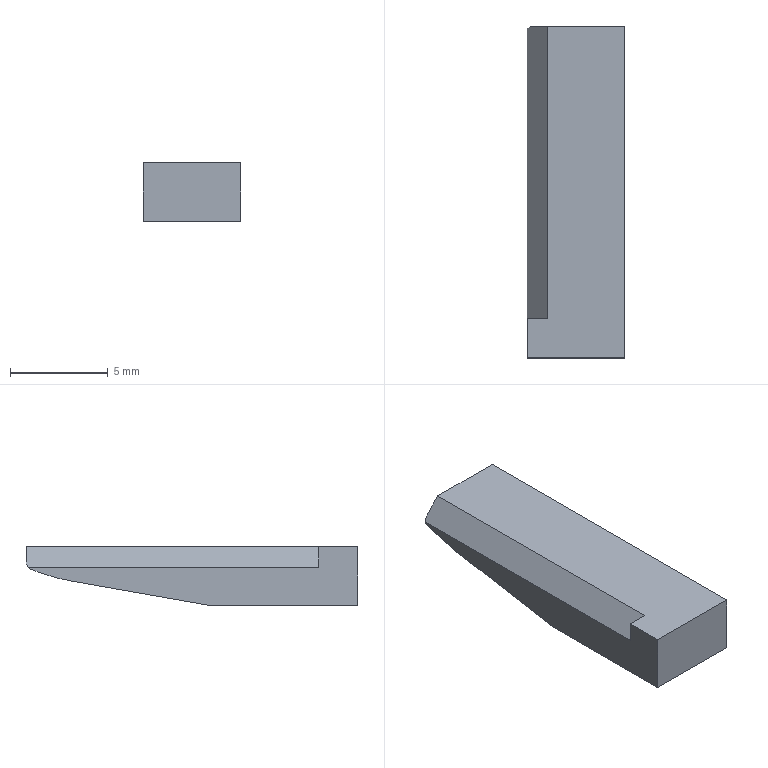Component | SolidWorks | 04LowerMaterialReceivingSwingAngleAssembly(3920)-1_04LowerMaterialReceivingDieAssembly(3920)-1_H2020022-0446-1(3920)-2 | 1 solid | 12 faces | box 5 x 17 x 3 mm | volume 207 mm3 | plane 10 | cylinder 2 | commonest cylinder face diameters 20 x1 1 x1 | material 45#Steel
build123d program:
from build123d import *

# Parameters (mm, degrees)
SKETCH1_W           = 5
SKETCH1_H           = 3
BOSS_EXTRUDE1_DEPTH = 17
CUT_EXTRUDE1_DEPTH  = 18.972
CUT_EXTRUDE2_DEPTH  = 18.972
FILLET2_R           = 10
FILLET3_R           = 0.5
CUT_EXTRUDE3_DEPTH  = 15


with BuildPart() as part:
    # Sketch1 → Boss-Extrude1 (new body)
    with BuildSketch(Plane(origin=(0, 0, 0), x_dir=(1, 0, 0), z_dir=(0, 1, 0))):
        with Locations((2.5, 1.5)):
            Rectangle(SKETCH1_W, SKETCH1_H)
    extrude(amount=BOSS_EXTRUDE1_DEPTH)

    # Sketch2 → Cut-Extrude1 (cut, through all)
    with BuildSketch(Plane.ZY):
        Polygon((-3, 7.65), (-1.351, 17), (-3, 17), align=None)
    extrude(amount=-CUT_EXTRUDE1_DEPTH, mode=Mode.SUBTRACT)

    # Sketch3 → Cut-Extrude2 (cut, through all)
    with BuildSketch(Plane.ZY):
        Polygon((-1.616, 15.5), (-1.07, 17), (-1.351, 17), align=None)
    extrude(amount=-CUT_EXTRUDE2_DEPTH, mode=Mode.SUBTRACT)

    # Fillet2
    fillet2_edges = [part.edges().sort_by_distance(p)[0] for p in [
        (2.5, 15.5, -1.616),
    ]]
    fillet(fillet2_edges, radius=FILLET2_R)

    # Fillet3
    fillet3_edges = [part.edges().sort_by_distance(p)[0] for p in [
        (2.5, 17, -1.07),
    ]]
    fillet(fillet3_edges, radius=FILLET3_R)

    # Sketch4 → Cut-Extrude3 (cut)
    with BuildSketch(Plane(origin=(0, 17, 0), x_dir=(1, 0, 0), z_dir=(0, 1, 0))):
        Polygon((0, 0), (0, 1.05), (1.05, 0), align=None)
    extrude(amount=-CUT_EXTRUDE3_DEPTH, mode=Mode.SUBTRACT)


solid = part.part

# Placed as in the assembly
solid = solid.moved(Location((-2.459, 271.013, 299.909), (0, 0, 0)))
STEP:
#1=COLOUR_RGB('',0.7922,0.8196,0.9333);
#2=FILL_AREA_STYLE_COLOUR('',#1);
#3=FILL_AREA_STYLE('',(#2));
#4=SURFACE_STYLE_FILL_AREA(#3);
#5=SURFACE_SIDE_STYLE('',(#4));
#6=SURFACE_STYLE_USAGE(.BOTH.,#5);
#7=PRESENTATION_STYLE_ASSIGNMENT((#6));
#8=CARTESIAN_POINT('',(-0.09682,10.749,11.766));
#9=VERTEX_POINT('',#8);
#10=CARTESIAN_POINT('',(-0.09682,10.749,11.807));
#11=VERTEX_POINT('',#10);
#12=CARTESIAN_POINT('',(-0.09682,10.749,11.807));
#13=DIRECTION('',(0.,0.,1.));
#14=VECTOR('',#13,39.37);
#15=LINE('',#12,#14);
#16=EDGE_CURVE('',#9,#11,#15,.T.);
#17=ORIENTED_EDGE('',*,*,#16,.F.);
#18=CARTESIAN_POINT('',(-0.09682,11.334,11.766));
#19=VERTEX_POINT('',#18);
#20=CARTESIAN_POINT('',(-0.09682,10.749,11.766));
#21=DIRECTION('',(0.,1.,0.));
#22=VECTOR('',#21,39.37);
#23=LINE('',#20,#22);
#24=EDGE_CURVE('',#9,#19,#23,.T.);
#25=ORIENTED_EDGE('',*,*,#24,.T.);
#26=CARTESIAN_POINT('',(-0.09682,11.326,11.761));
#27=VERTEX_POINT('',#26);
#28=CARTESIAN_POINT('',(-0.09682,11.319,11.779));
#29=DIRECTION('',(-1.,0.,0.));
#30=DIRECTION('',(0.,0.,-1.));
#31=AXIS2_PLACEMENT_3D('',#28,#29,#30);
#32=CIRCLE('',#31,0.01969);
#33=EDGE_CURVE('',#19,#27,#32,.T.);
#34=ORIENTED_EDGE('',*,*,#33,.T.);
#35=CARTESIAN_POINT('',(-0.09682,11.312,11.756));
#36=VERTEX_POINT('',#35);
#37=CARTESIAN_POINT('',(-0.09682,11.28,11.744));
#38=DIRECTION('',(0.,0.9397,0.342));
#39=VECTOR('',#38,39.37);
#40=LINE('',#37,#39);
#41=EDGE_CURVE('',#36,#27,#40,.T.);
#42=ORIENTED_EDGE('',*,*,#41,.F.);
#43=CARTESIAN_POINT('',(-0.09682,11.246,11.738));
#44=VERTEX_POINT('',#43);
#45=CARTESIAN_POINT('',(-0.09682,11.178,12.126));
#46=DIRECTION('',(-1.,0.,0.));
#47=DIRECTION('',(0.,-0.,-1.));
#48=AXIS2_PLACEMENT_3D('',#45,#46,#47);
#49=CIRCLE('',#48,0.3937);
#50=EDGE_CURVE('',#36,#44,#49,.T.);
#51=ORIENTED_EDGE('',*,*,#50,.T.);
#52=CARTESIAN_POINT('',(-0.09682,10.971,11.689));
#53=VERTEX_POINT('',#52);
#54=CARTESIAN_POINT('',(-0.09682,10.971,11.689));
#55=DIRECTION('',(0.,0.9848,0.1736));
#56=VECTOR('',#55,39.37);
#57=LINE('',#54,#56);
#58=EDGE_CURVE('',#53,#44,#57,.T.);
#59=ORIENTED_EDGE('',*,*,#58,.F.);
#60=CARTESIAN_POINT('',(-0.09682,10.67,11.689));
#61=VERTEX_POINT('',#60);
#62=CARTESIAN_POINT('',(-0.09682,11.339,11.689));
#63=DIRECTION('',(0.,-1.,0.));
#64=VECTOR('',#63,39.37);
#65=LINE('',#62,#64);
#66=EDGE_CURVE('',#53,#61,#65,.T.);
#67=ORIENTED_EDGE('',*,*,#66,.T.);
#68=CARTESIAN_POINT('',(-0.09682,10.67,11.807));
#69=VERTEX_POINT('',#68);
#70=CARTESIAN_POINT('',(-0.09682,10.67,11.807));
#71=DIRECTION('',(0.,0.,1.));
#72=VECTOR('',#71,39.37);
#73=LINE('',#70,#72);
#74=EDGE_CURVE('',#61,#69,#73,.T.);
#75=ORIENTED_EDGE('',*,*,#74,.T.);
#76=CARTESIAN_POINT('',(-0.09682,11.339,11.807));
#77=DIRECTION('',(0.,-1.,0.));
#78=VECTOR('',#77,39.37);
#79=LINE('',#76,#78);
#80=EDGE_CURVE('',#11,#69,#79,.T.);
#81=ORIENTED_EDGE('',*,*,#80,.F.);
#82=EDGE_LOOP('',(#17,#25,#34,#42,#51,#59,#67,#75,#81));
#83=FACE_OUTER_BOUND('',#82,.T.);
#84=CARTESIAN_POINT('',(-0.09682,11.339,11.807));
#85=DIRECTION('',(1.,0.,0.));
#86=DIRECTION('',(0.,0.,-1.));
#87=AXIS2_PLACEMENT_3D('',#84,#85,#86);
#88=PLANE('',#87);
#89=ADVANCED_FACE('',(#83),#88,.F.);
#90=CARTESIAN_POINT('',(-0.05548,11.339,11.807));
#91=VERTEX_POINT('',#90);
#92=CARTESIAN_POINT('',(0.1,11.339,11.807));
#93=VERTEX_POINT('',#92);
#94=CARTESIAN_POINT('',(-0.09682,11.339,11.807));
#95=DIRECTION('',(1.,0.,0.));
#96=VECTOR('',#95,39.37);
#97=LINE('',#94,#96);
#98=EDGE_CURVE('',#91,#93,#97,.T.);
#99=ORIENTED_EDGE('',*,*,#98,.F.);
#100=CARTESIAN_POINT('',(-0.05548,10.749,11.807));
#101=VERTEX_POINT('',#100);
#102=CARTESIAN_POINT('',(-0.05548,10.749,11.807));
#103=DIRECTION('',(0.,1.,0.));
#104=VECTOR('',#103,39.37);
#105=LINE('',#102,#104);
#106=EDGE_CURVE('',#101,#91,#105,.T.);
#107=ORIENTED_EDGE('',*,*,#106,.F.);
#108=CARTESIAN_POINT('',(-0.05548,10.749,11.807));
#109=DIRECTION('',(1.,0.,0.));
#110=VECTOR('',#109,39.37);
#111=LINE('',#108,#110);
#112=EDGE_CURVE('',#11,#101,#111,.T.);
#113=ORIENTED_EDGE('',*,*,#112,.F.);
#114=ORIENTED_EDGE('',*,*,#80,.T.);
#115=CARTESIAN_POINT('',(0.1,10.67,11.807));
#116=VERTEX_POINT('',#115);
#117=CARTESIAN_POINT('',(-0.09682,10.67,11.807));
#118=DIRECTION('',(1.,0.,0.));
#119=VECTOR('',#118,39.37);
#120=LINE('',#117,#119);
#121=EDGE_CURVE('',#69,#116,#120,.T.);
#122=ORIENTED_EDGE('',*,*,#121,.T.);
#123=CARTESIAN_POINT('',(0.1,11.339,11.807));
#124=DIRECTION('',(0.,-1.,0.));
#125=VECTOR('',#124,39.37);
#126=LINE('',#123,#125);
#127=EDGE_CURVE('',#93,#116,#126,.T.);
#128=ORIENTED_EDGE('',*,*,#127,.F.);
#129=EDGE_LOOP('',(#99,#107,#113,#114,#122,#128));
#130=FACE_OUTER_BOUND('',#129,.T.);
#131=CARTESIAN_POINT('',(-0.09682,11.339,11.807));
#132=DIRECTION('',(0.,0.,-1.));
#133=DIRECTION('',(-1.,0.,0.));
#134=AXIS2_PLACEMENT_3D('',#131,#132,#133);
#135=PLANE('',#134);
#136=ADVANCED_FACE('',(#130),#135,.F.);
#137=CARTESIAN_POINT('',(0.1,11.312,11.756));
#138=VERTEX_POINT('',#137);
#139=CARTESIAN_POINT('',(0.1,11.326,11.761));
#140=VERTEX_POINT('',#139);
#141=CARTESIAN_POINT('',(0.1,11.28,11.744));
#142=DIRECTION('',(0.,0.9397,0.342));
#143=VECTOR('',#142,39.37);
#144=LINE('',#141,#143);
#145=EDGE_CURVE('',#138,#140,#144,.T.);
#146=ORIENTED_EDGE('',*,*,#145,.T.);
#147=CARTESIAN_POINT('',(0.1,11.339,11.779));
#148=VERTEX_POINT('',#147);
#149=CARTESIAN_POINT('',(0.1,11.319,11.779));
#150=DIRECTION('',(1.,0.,0.));
#151=DIRECTION('',(0.,0.,1.));
#152=AXIS2_PLACEMENT_3D('',#149,#150,#151);
#153=CIRCLE('',#152,0.01969);
#154=EDGE_CURVE('',#140,#148,#153,.T.);
#155=ORIENTED_EDGE('',*,*,#154,.T.);
#156=CARTESIAN_POINT('',(0.1,11.339,11.807));
#157=DIRECTION('',(0.,0.,-1.));
#158=VECTOR('',#157,39.37);
#159=LINE('',#156,#158);
#160=EDGE_CURVE('',#93,#148,#159,.T.);
#161=ORIENTED_EDGE('',*,*,#160,.F.);
#162=ORIENTED_EDGE('',*,*,#127,.T.);
#163=CARTESIAN_POINT('',(0.1,10.67,11.689));
#164=VERTEX_POINT('',#163);
#165=CARTESIAN_POINT('',(0.1,10.67,11.807));
#166=DIRECTION('',(0.,0.,-1.));
#167=VECTOR('',#166,39.37);
#168=LINE('',#165,#167);
#169=EDGE_CURVE('',#116,#164,#168,.T.);
#170=ORIENTED_EDGE('',*,*,#169,.T.);
#171=CARTESIAN_POINT('',(0.1,10.971,11.689));
#172=VERTEX_POINT('',#171);
#173=CARTESIAN_POINT('',(0.1,11.339,11.689));
#174=DIRECTION('',(0.,-1.,0.));
#175=VECTOR('',#174,39.37);
#176=LINE('',#173,#175);
#177=EDGE_CURVE('',#172,#164,#176,.T.);
#178=ORIENTED_EDGE('',*,*,#177,.F.);
#179=CARTESIAN_POINT('',(0.1,11.246,11.738));
#180=VERTEX_POINT('',#179);
#181=CARTESIAN_POINT('',(0.1,10.971,11.689));
#182=DIRECTION('',(0.,0.9848,0.1736));
#183=VECTOR('',#182,39.37);
#184=LINE('',#181,#183);
#185=EDGE_CURVE('',#172,#180,#184,.T.);
#186=ORIENTED_EDGE('',*,*,#185,.T.);
#187=CARTESIAN_POINT('',(0.1,11.178,12.126));
#188=DIRECTION('',(1.,0.,0.));
#189=DIRECTION('',(0.,0.,1.));
#190=AXIS2_PLACEMENT_3D('',#187,#188,#189);
#191=CIRCLE('',#190,0.3937);
#192=EDGE_CURVE('',#180,#138,#191,.T.);
#193=ORIENTED_EDGE('',*,*,#192,.T.);
#194=EDGE_LOOP('',(#146,#155,#161,#162,#170,#178,#186,#193));
#195=FACE_OUTER_BOUND('',#194,.T.);
#196=CARTESIAN_POINT('',(0.1,11.339,11.807));
#197=DIRECTION('',(-1.,0.,0.));
#198=DIRECTION('',(0.,0.,1.));
#199=AXIS2_PLACEMENT_3D('',#196,#197,#198);
#200=PLANE('',#199);
#201=ADVANCED_FACE('',(#195),#200,.F.);
#202=ORIENTED_EDGE('',*,*,#66,.F.);
#203=CARTESIAN_POINT('',(0.1,10.971,11.689));
#204=DIRECTION('',(-1.,0.,0.));
#205=VECTOR('',#204,39.37);
#206=LINE('',#203,#205);
#207=EDGE_CURVE('',#172,#53,#206,.T.);
#208=ORIENTED_EDGE('',*,*,#207,.F.);
#209=ORIENTED_EDGE('',*,*,#177,.T.);
#210=CARTESIAN_POINT('',(-0.09682,10.67,11.689));
#211=DIRECTION('',(-1.,0.,0.));
#212=VECTOR('',#211,39.37);
#213=LINE('',#210,#212);
#214=EDGE_CURVE('',#164,#61,#213,.T.);
#215=ORIENTED_EDGE('',*,*,#214,.T.);
#216=EDGE_LOOP('',(#202,#208,#209,#215));
#217=FACE_OUTER_BOUND('',#216,.T.);
#218=CARTESIAN_POINT('',(-0.09682,11.339,11.689));
#219=DIRECTION('',(0.,0.,1.));
#220=DIRECTION('',(1.,0.,0.));
#221=AXIS2_PLACEMENT_3D('',#218,#219,#220);
#222=PLANE('',#221);
#223=ADVANCED_FACE('',(#217),#222,.F.);
#224=CARTESIAN_POINT('',(-0.08382,11.339,11.779));
#225=VERTEX_POINT('',#224);
#226=CARTESIAN_POINT('',(-0.09682,11.339,11.779));
#227=DIRECTION('',(-1.,0.,0.));
#228=VECTOR('',#227,39.37);
#229=LINE('',#226,#228);
#230=EDGE_CURVE('',#148,#225,#229,.T.);
#231=ORIENTED_EDGE('',*,*,#230,.T.);
#232=CARTESIAN_POINT('',(-0.09682,11.339,11.766));
#233=DIRECTION('',(-0.7071,0.,-0.7071));
#234=VECTOR('',#233,39.37);
#235=LINE('',#232,#234);
#236=EDGE_CURVE('',#91,#225,#235,.T.);
#237=ORIENTED_EDGE('',*,*,#236,.F.);
#238=ORIENTED_EDGE('',*,*,#98,.T.);
#239=ORIENTED_EDGE('',*,*,#160,.T.);
#240=EDGE_LOOP('',(#231,#237,#238,#239));
#241=FACE_OUTER_BOUND('',#240,.T.);
#242=CARTESIAN_POINT('',(-0.09682,11.339,11.807));
#243=DIRECTION('',(0.,-1.,0.));
#244=DIRECTION('',(0.,0.,-1.));
#245=AXIS2_PLACEMENT_3D('',#242,#243,#244);
#246=PLANE('',#245);
#247=ADVANCED_FACE('',(#241),#246,.F.);
#248=ORIENTED_EDGE('',*,*,#74,.F.);
#249=ORIENTED_EDGE('',*,*,#214,.F.);
#250=ORIENTED_EDGE('',*,*,#169,.F.);
#251=ORIENTED_EDGE('',*,*,#121,.F.);
#252=EDGE_LOOP('',(#248,#249,#250,#251));
#253=FACE_OUTER_BOUND('',#252,.T.);
#254=CARTESIAN_POINT('',(-0.09682,10.67,11.807));
#255=DIRECTION('',(0.,-1.,0.));
#256=DIRECTION('',(0.,0.,-1.));
#257=AXIS2_PLACEMENT_3D('',#254,#255,#256);
#258=PLANE('',#257);
#259=ADVANCED_FACE('',(#253),#258,.T.);
#260=ORIENTED_EDGE('',*,*,#58,.T.);
#261=CARTESIAN_POINT('',(0.1,11.246,11.738));
#262=DIRECTION('',(1.,0.,0.));
#263=VECTOR('',#262,39.37);
#264=LINE('',#261,#263);
#265=EDGE_CURVE('',#44,#180,#264,.T.);
#266=ORIENTED_EDGE('',*,*,#265,.T.);
#267=ORIENTED_EDGE('',*,*,#185,.F.);
#268=ORIENTED_EDGE('',*,*,#207,.T.);
#269=EDGE_LOOP('',(#260,#266,#267,#268));
#270=FACE_OUTER_BOUND('',#269,.T.);
#271=CARTESIAN_POINT('',(0.1,10.971,11.689));
#272=DIRECTION('',(0.,-0.1736,0.9848));
#273=DIRECTION('',(0.,-0.9848,-0.1736));
#274=AXIS2_PLACEMENT_3D('',#271,#272,#273);
#275=PLANE('',#274);
#276=ADVANCED_FACE('',(#270),#275,.F.);
#277=ORIENTED_EDGE('',*,*,#41,.T.);
#278=CARTESIAN_POINT('',(0.1,11.326,11.761));
#279=DIRECTION('',(1.,0.,0.));
#280=VECTOR('',#279,39.37);
#281=LINE('',#278,#280);
#282=EDGE_CURVE('',#27,#140,#281,.T.);
#283=ORIENTED_EDGE('',*,*,#282,.T.);
#284=ORIENTED_EDGE('',*,*,#145,.F.);
#285=CARTESIAN_POINT('',(0.1,11.312,11.756));
#286=DIRECTION('',(-1.,0.,0.));
#287=VECTOR('',#286,39.37);
#288=LINE('',#285,#287);
#289=EDGE_CURVE('',#138,#36,#288,.T.);
#290=ORIENTED_EDGE('',*,*,#289,.T.);
#291=EDGE_LOOP('',(#277,#283,#284,#290));
#292=FACE_OUTER_BOUND('',#291,.T.);
#293=CARTESIAN_POINT('',(0.1,11.28,11.744));
#294=DIRECTION('',(0.,-0.342,0.9397));
#295=DIRECTION('',(0.,-0.9397,-0.342));
#296=AXIS2_PLACEMENT_3D('',#293,#294,#295);
#297=PLANE('',#296);
#298=ADVANCED_FACE('',(#292),#297,.F.);
#299=ORIENTED_EDGE('',*,*,#192,.F.);
#300=ORIENTED_EDGE('',*,*,#265,.F.);
#301=ORIENTED_EDGE('',*,*,#50,.F.);
#302=ORIENTED_EDGE('',*,*,#289,.F.);
#303=EDGE_LOOP('',(#299,#300,#301,#302));
#304=FACE_OUTER_BOUND('',#303,.T.);
#305=CARTESIAN_POINT('',(0.1,11.178,12.126));
#306=DIRECTION('',(-1.,0.,0.));
#307=DIRECTION('',(0.,0.,1.));
#308=AXIS2_PLACEMENT_3D('',#305,#306,#307);
#309=CYLINDRICAL_SURFACE('',#308,0.3937);
#310=ADVANCED_FACE('',(#304),#309,.T.);
#311=CARTESIAN_POINT('',(-0.08382,11.339,11.779));
#312=CARTESIAN_POINT('',(-0.08866,11.339,11.774));
#313=CARTESIAN_POINT('',(-0.09319,11.337,11.77));
#314=CARTESIAN_POINT('',(-0.09682,11.334,11.766));
#315=(BOUNDED_CURVE()B_SPLINE_CURVE(3,(#311,#312,#313,#314),.UNSPECIFIED.,.F.,.T.)B_SPLINE_CURVE_WITH_KNOTS((4,4),(4.712,5.434),.UNSPECIFIED.)CURVE()GEOMETRIC_REPRESENTATION_ITEM()RATIONAL_B_SPLINE_CURVE((1.,0.9571,0.9571,1.))REPRESENTATION_ITEM(''));
#316=EDGE_CURVE('',#225,#19,#315,.T.);
#317=ORIENTED_EDGE('',*,*,#316,.F.);
#318=ORIENTED_EDGE('',*,*,#230,.F.);
#319=ORIENTED_EDGE('',*,*,#154,.F.);
#320=ORIENTED_EDGE('',*,*,#282,.F.);
#321=ORIENTED_EDGE('',*,*,#33,.F.);
#322=EDGE_LOOP('',(#317,#318,#319,#320,#321));
#323=FACE_OUTER_BOUND('',#322,.T.);
#324=CARTESIAN_POINT('',(-0.09682,11.319,11.779));
#325=DIRECTION('',(-1.,0.,0.));
#326=DIRECTION('',(0.,0.,1.));
#327=AXIS2_PLACEMENT_3D('',#324,#325,#326);
#328=CYLINDRICAL_SURFACE('',#327,0.01969);
#329=ADVANCED_FACE('',(#323),#328,.T.);
#330=ORIENTED_EDGE('',*,*,#316,.T.);
#331=ORIENTED_EDGE('',*,*,#24,.F.);
#332=CARTESIAN_POINT('',(-0.09682,10.749,11.766));
#333=DIRECTION('',(-0.7071,0.,-0.7071));
#334=VECTOR('',#333,39.37);
#335=LINE('',#332,#334);
#336=EDGE_CURVE('',#101,#9,#335,.T.);
#337=ORIENTED_EDGE('',*,*,#336,.F.);
#338=ORIENTED_EDGE('',*,*,#106,.T.);
#339=ORIENTED_EDGE('',*,*,#236,.T.);
#340=EDGE_LOOP('',(#330,#331,#337,#338,#339));
#341=FACE_OUTER_BOUND('',#340,.T.);
#342=CARTESIAN_POINT('',(-0.09682,10.749,11.766));
#343=DIRECTION('',(0.7071,0.,-0.7071));
#344=DIRECTION('',(-0.7071,0.,-0.7071));
#345=AXIS2_PLACEMENT_3D('',#342,#343,#344);
#346=PLANE('',#345);
#347=ADVANCED_FACE('',(#341),#346,.F.);
#348=ORIENTED_EDGE('',*,*,#112,.T.);
#349=ORIENTED_EDGE('',*,*,#336,.T.);
#350=ORIENTED_EDGE('',*,*,#16,.T.);
#351=EDGE_LOOP('',(#348,#349,#350));
#352=FACE_OUTER_BOUND('',#351,.T.);
#353=CARTESIAN_POINT('',(-0.09682,10.749,11.807));
#354=DIRECTION('',(0.,-1.,0.));
#355=DIRECTION('',(0.,0.,-1.));
#356=AXIS2_PLACEMENT_3D('',#353,#354,#355);
#357=PLANE('',#356);
#358=ADVANCED_FACE('',(#352),#357,.F.);
#359=CLOSED_SHELL('',(#89,#136,#201,#223,#247,#259,#276,#298,#310,#329,#347,#358));
#360=MANIFOLD_SOLID_BREP('',#359);
#361=STYLED_ITEM('',(#7),#360);
#362=PRESENTATION_LAYER_ASSIGNMENT('','',(#361));
#363=(LENGTH_UNIT()NAMED_UNIT(*)SI_UNIT($,.METRE.));
#364=LENGTH_MEASURE_WITH_UNIT(LENGTH_MEASURE(0.0254),#363);
#365=DIMENSIONAL_EXPONENTS(1.,0.,0.,0.,0.,0.,0.);
#366=(CONVERSION_BASED_UNIT('',#364)LENGTH_UNIT()NAMED_UNIT(#365));
#367=UNCERTAINTY_MEASURE_WITH_UNIT(LENGTH_MEASURE(0.00001),#366,'','');
#368=(NAMED_UNIT(*)PLANE_ANGLE_UNIT()SI_UNIT($,.RADIAN.));
#369=(NAMED_UNIT(*)SI_UNIT($,.STERADIAN.)SOLID_ANGLE_UNIT());
#370=(GEOMETRIC_REPRESENTATION_CONTEXT(3)GLOBAL_UNCERTAINTY_ASSIGNED_CONTEXT((#367))GLOBAL_UNIT_ASSIGNED_CONTEXT((#366,#368,#369))REPRESENTATION_CONTEXT('',''));
#371=MECHANICAL_DESIGN_GEOMETRIC_PRESENTATION_REPRESENTATION('',(#361),#370);
#372=CARTESIAN_POINT('',(0.,0.,0.));
#373=DIRECTION('',(0.,0.,1.));
#374=DIRECTION('',(1.,0.,0.));
#375=AXIS2_PLACEMENT_3D('',#372,#373,#374);
#376=(LENGTH_UNIT()NAMED_UNIT(*)SI_UNIT($,.METRE.));
#377=LENGTH_MEASURE_WITH_UNIT(LENGTH_MEASURE(0.0254),#376);
#378=DIMENSIONAL_EXPONENTS(1.,0.,0.,0.,0.,0.,0.);
#379=(CONVERSION_BASED_UNIT('',#377)LENGTH_UNIT()NAMED_UNIT(#378));
#380=UNCERTAINTY_MEASURE_WITH_UNIT(LENGTH_MEASURE(0.00001),#379,'','');
#381=(NAMED_UNIT(*)PLANE_ANGLE_UNIT()SI_UNIT($,.RADIAN.));
#382=(NAMED_UNIT(*)SI_UNIT($,.STERADIAN.)SOLID_ANGLE_UNIT());
#383=(GEOMETRIC_REPRESENTATION_CONTEXT(3)GLOBAL_UNCERTAINTY_ASSIGNED_CONTEXT((#380))GLOBAL_UNIT_ASSIGNED_CONTEXT((#379,#381,#382))REPRESENTATION_CONTEXT('',''));
#384=ADVANCED_BREP_SHAPE_REPRESENTATION('',(#360,#375),#383);